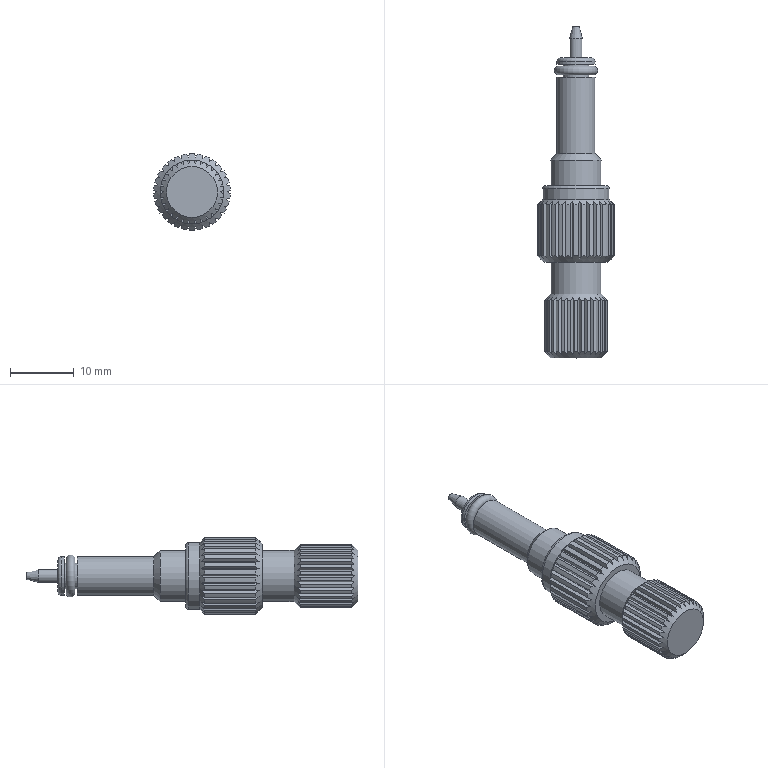Component | NX | ADJUSTMENT_KNOB | 2 solids | 203 faces | volume 2876 mm3 | plane 127 | cylinder 67 | cone 6 | torus 3 | commonest cylinder face diameters 12 x30 10 x30 6 x2 8 x2 2 x1 4 x1 10.5 x1